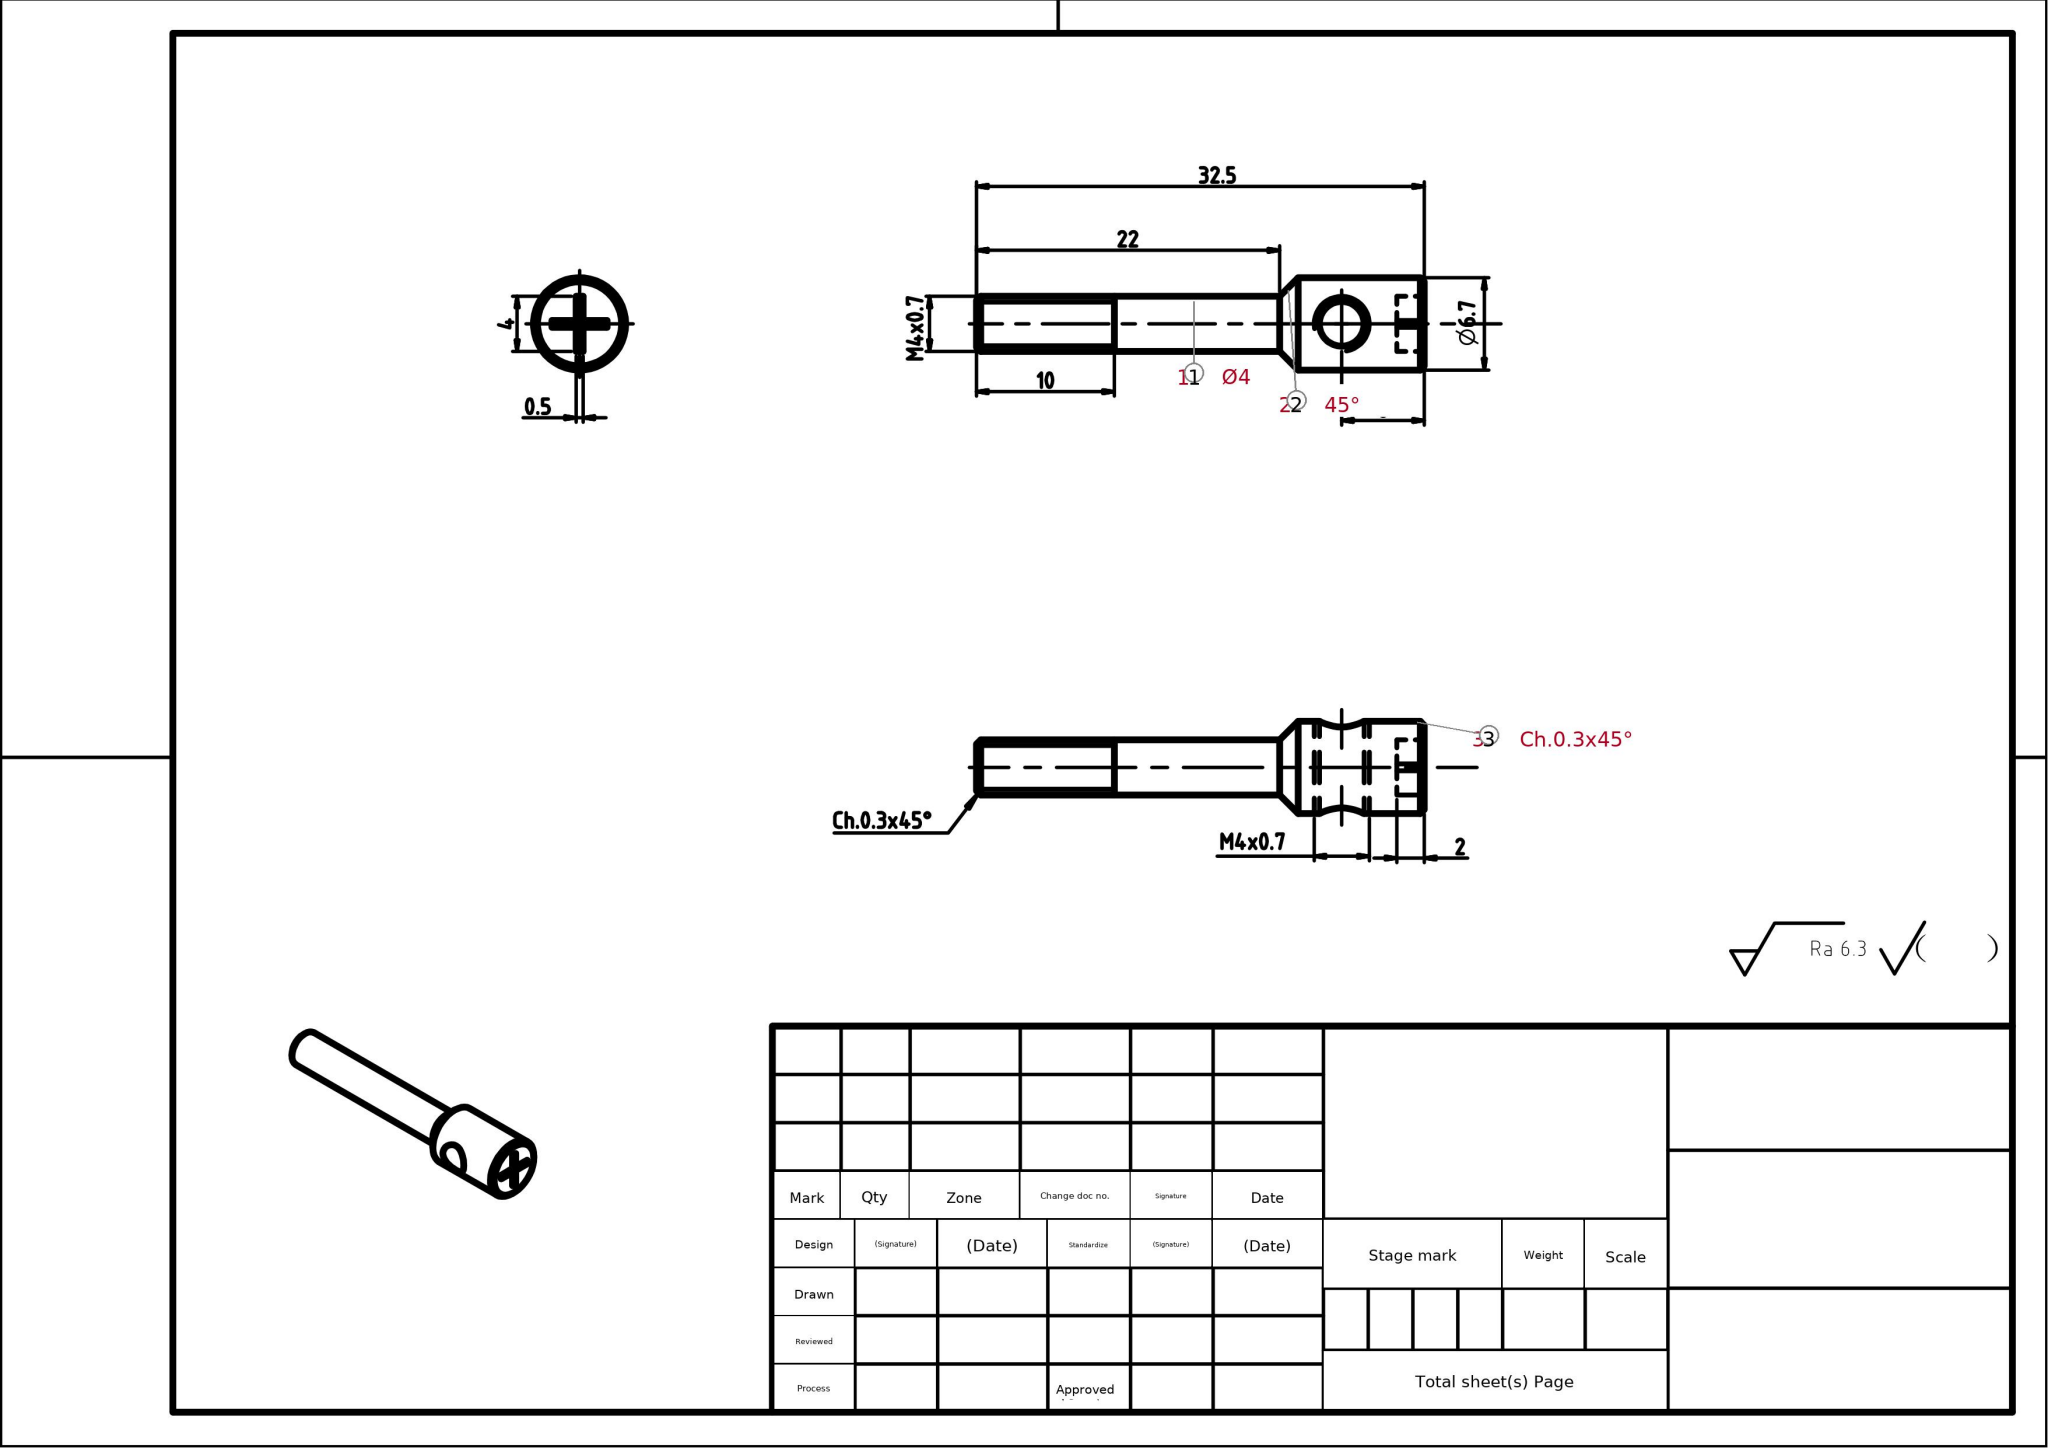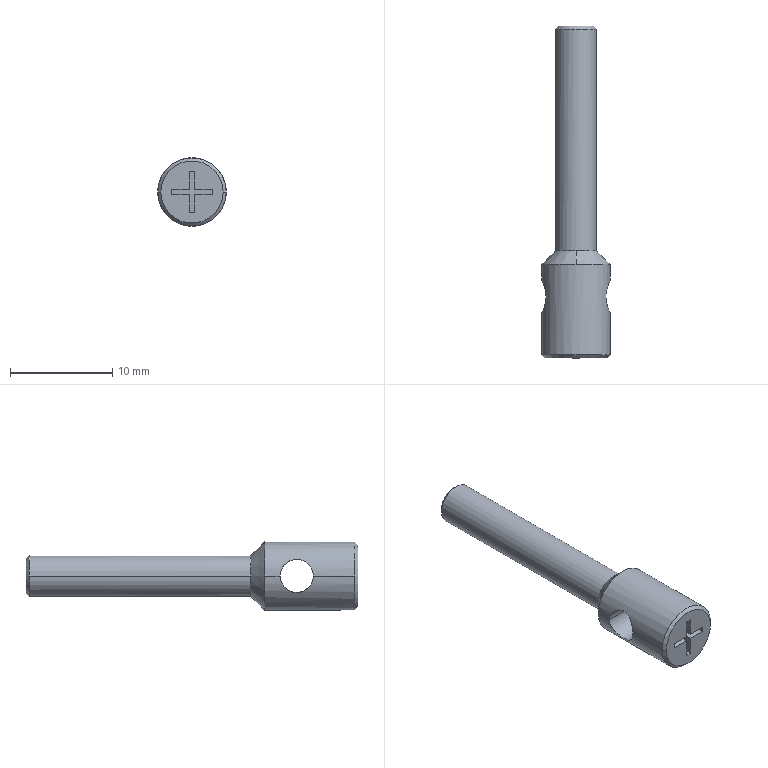Part | SolidWorks | mm | 1 solid | 27 faces | box 6.7 x 32.5 x 6.7 mm | volume 567 mm3 | plane 15 | cone 6 | cylinder 6 | commonest cylinder face diameters 3.242 x2 6.7 x2 4 x2
STEP:
#1=CARTESIAN_POINT('',(0.,10.5,2.));
#2=VERTEX_POINT('',#1);
#3=CARTESIAN_POINT('',(2.,10.5,-0.));
#4=VERTEX_POINT('',#3);
#5=CARTESIAN_POINT('',(0.,10.5,0.));
#6=DIRECTION('',(0.,1.,0.));
#7=DIRECTION('',(-1.,0.,0.));
#8=AXIS2_PLACEMENT_3D('',#5,#6,#7);
#9=CIRCLE('',#8,2.);
#10=EDGE_CURVE('',#2,#4,#9,.T.);
#11=ORIENTED_EDGE('',*,*,#10,.F.);
#12=CARTESIAN_POINT('',(0.,9.15,3.35));
#13=VERTEX_POINT('',#12);
#14=CARTESIAN_POINT('',(0.,9.825,2.675));
#15=DIRECTION('',(0.,-0.7071,0.7071));
#16=VECTOR('',#15,1000.);
#17=LINE('',#14,#16);
#18=EDGE_CURVE('',#2,#13,#17,.T.);
#19=ORIENTED_EDGE('',*,*,#18,.T.);
#20=CARTESIAN_POINT('',(3.35,9.15,0.));
#21=VERTEX_POINT('',#20);
#22=CARTESIAN_POINT('',(0.,9.15,0.));
#23=DIRECTION('',(0.,-1.,0.));
#24=DIRECTION('',(-1.,0.,0.));
#25=AXIS2_PLACEMENT_3D('',#22,#23,#24);
#26=CIRCLE('',#25,3.35);
#27=EDGE_CURVE('',#21,#13,#26,.T.);
#28=ORIENTED_EDGE('',*,*,#27,.F.);
#29=CARTESIAN_POINT('',(0.,9.15,-3.35));
#30=VERTEX_POINT('',#29);
#31=CARTESIAN_POINT('',(0.,9.15,0.));
#32=DIRECTION('',(0.,-1.,0.));
#33=DIRECTION('',(-1.,0.,0.));
#34=AXIS2_PLACEMENT_3D('',#31,#32,#33);
#35=CIRCLE('',#34,3.35);
#36=EDGE_CURVE('',#30,#21,#35,.T.);
#37=ORIENTED_EDGE('',*,*,#36,.F.);
#38=CARTESIAN_POINT('',(0.,10.5,-2.));
#39=VERTEX_POINT('',#38);
#40=CARTESIAN_POINT('',(0.,9.825,-2.675));
#41=DIRECTION('',(0.,-0.7071,-0.7071));
#42=VECTOR('',#41,1000.);
#43=LINE('',#40,#42);
#44=EDGE_CURVE('',#39,#30,#43,.T.);
#45=ORIENTED_EDGE('',*,*,#44,.F.);
#46=CARTESIAN_POINT('',(0.,10.5,0.));
#47=DIRECTION('',(0.,1.,0.));
#48=DIRECTION('',(-1.,0.,0.));
#49=AXIS2_PLACEMENT_3D('',#46,#47,#48);
#50=CIRCLE('',#49,2.);
#51=EDGE_CURVE('',#4,#39,#50,.T.);
#52=ORIENTED_EDGE('',*,*,#51,.F.);
#53=EDGE_LOOP('',(#11,#19,#28,#37,#45,#52));
#54=FACE_OUTER_BOUND('',#53,.T.);
#55=CARTESIAN_POINT('',(0.,9.825,0.));
#56=DIRECTION('',(0.,-1.,0.));
#57=DIRECTION('',(0.,0.,-1.));
#58=AXIS2_PLACEMENT_3D('',#55,#56,#57);
#59=CONICAL_SURFACE('',#58,2.675,0.7854);
#60=ADVANCED_FACE('',(#54),#59,.T.);
#61=CARTESIAN_POINT('',(-3.35,4.379,0.));
#62=VERTEX_POINT('',#61);
#63=CARTESIAN_POINT('',(-3.35,7.621,0.));
#64=VERTEX_POINT('',#63);
#65=CARTESIAN_POINT('',(-3.35,4.379,0.));
#66=CARTESIAN_POINT('',(-3.35,4.379,-0.1079));
#67=CARTESIAN_POINT('',(-3.345,4.389,-0.2144));
#68=CARTESIAN_POINT('',(-3.325,4.431,-0.4232));
#69=CARTESIAN_POINT('',(-3.31,4.463,-0.5273));
#70=CARTESIAN_POINT('',(-3.272,4.546,-0.7243));
#71=CARTESIAN_POINT('',(-3.25,4.596,-0.817));
#72=CARTESIAN_POINT('',(-3.201,4.712,-0.9908));
#73=CARTESIAN_POINT('',(-3.175,4.778,-1.071));
#74=CARTESIAN_POINT('',(-3.12,4.931,-1.224));
#75=CARTESIAN_POINT('',(-3.092,5.013,-1.291));
#76=CARTESIAN_POINT('',(-3.054,5.143,-1.377));
#77=CARTESIAN_POINT('',(-3.042,5.188,-1.404));
#78=CARTESIAN_POINT('',(-3.018,5.28,-1.453));
#79=CARTESIAN_POINT('',(-3.008,5.325,-1.475));
#80=CARTESIAN_POINT('',(-2.955,5.577,-1.58));
#81=CARTESIAN_POINT('',(-2.932,5.786,-1.621));
#82=CARTESIAN_POINT('',(-2.932,6.107,-1.621));
#83=CARTESIAN_POINT('',(-2.937,6.213,-1.611));
#84=CARTESIAN_POINT('',(-2.954,6.369,-1.58));
#85=CARTESIAN_POINT('',(-2.961,6.42,-1.567));
#86=CARTESIAN_POINT('',(-2.978,6.523,-1.535));
#87=CARTESIAN_POINT('',(-2.987,6.576,-1.516));
#88=CARTESIAN_POINT('',(-3.018,6.721,-1.455));
#89=CARTESIAN_POINT('',(-3.041,6.813,-1.406));
#90=CARTESIAN_POINT('',(-3.092,6.987,-1.291));
#91=CARTESIAN_POINT('',(-3.12,7.07,-1.223));
#92=CARTESIAN_POINT('',(-3.175,7.221,-1.072));
#93=CARTESIAN_POINT('',(-3.201,7.288,-0.9909));
#94=CARTESIAN_POINT('',(-3.25,7.404,-0.8171));
#95=CARTESIAN_POINT('',(-3.272,7.453,-0.7259));
#96=CARTESIAN_POINT('',(-3.329,7.579,-0.4256));
#97=CARTESIAN_POINT('',(-3.35,7.621,-0.2159));
#98=CARTESIAN_POINT('',(-3.35,7.621,0.));
#99=B_SPLINE_CURVE_WITH_KNOTS('',3,(#65,#66,#67,#68,#69,#70,#71,#72,#73,#74,#75,#76,#77,#78,#79,#80,#81,#82,#83,#84,#85,#86,#87,#88,#89,#90,#91,#92,#93,#94,#95,#96,#97,#98),.UNSPECIFIED.,.F.,.F.,(4,2,2,2,2,2,2,2,2,2,2,2,2,2,2,2,4),(0.,0.0625,0.125,0.1875,0.25,0.3125,0.3438,0.375,0.5,0.5625,0.5938,0.625,0.6875,0.75,0.8125,0.875,1.),.UNSPECIFIED.);
#100=EDGE_CURVE('',#62,#64,#99,.T.);
#101=ORIENTED_EDGE('',*,*,#100,.F.);
#102=CARTESIAN_POINT('',(3.35,4.379,-0.));
#103=VERTEX_POINT('',#102);
#104=CARTESIAN_POINT('',(30.503,4.379,0.));
#105=DIRECTION('',(1.,0.,0.));
#106=VECTOR('',#105,1000.);
#107=LINE('',#104,#106);
#108=EDGE_CURVE('',#62,#103,#107,.T.);
#109=ORIENTED_EDGE('',*,*,#108,.T.);
#110=CARTESIAN_POINT('',(2.932,6.,-1.621));
#111=VERTEX_POINT('',#110);
#112=CARTESIAN_POINT('',(2.932,6.,-1.621));
#113=CARTESIAN_POINT('',(2.932,5.893,-1.621));
#114=CARTESIAN_POINT('',(2.937,5.787,-1.611));
#115=CARTESIAN_POINT('',(2.954,5.631,-1.58));
#116=CARTESIAN_POINT('',(2.961,5.579,-1.567));
#117=CARTESIAN_POINT('',(2.978,5.477,-1.535));
#118=CARTESIAN_POINT('',(2.987,5.424,-1.516));
#119=CARTESIAN_POINT('',(3.018,5.279,-1.455));
#120=CARTESIAN_POINT('',(3.041,5.187,-1.406));
#121=CARTESIAN_POINT('',(3.092,5.013,-1.291));
#122=CARTESIAN_POINT('',(3.12,4.93,-1.223));
#123=CARTESIAN_POINT('',(3.175,4.779,-1.072));
#124=CARTESIAN_POINT('',(3.201,4.712,-0.9909));
#125=CARTESIAN_POINT('',(3.25,4.596,-0.8171));
#126=CARTESIAN_POINT('',(3.272,4.547,-0.7259));
#127=CARTESIAN_POINT('',(3.329,4.421,-0.4256));
#128=CARTESIAN_POINT('',(3.35,4.379,-0.2159));
#129=CARTESIAN_POINT('',(3.35,4.379,-0.));
#130=B_SPLINE_CURVE_WITH_KNOTS('',3,(#112,#113,#114,#115,#116,#117,#118,#119,#120,#121,#122,#123,#124,#125,#126,#127,#128,#129),.UNSPECIFIED.,.F.,.F.,(4,2,2,2,2,2,2,2,4),(0.,0.125,0.1875,0.25,0.375,0.5,0.625,0.75,1.),.UNSPECIFIED.);
#131=EDGE_CURVE('',#111,#103,#130,.T.);
#132=ORIENTED_EDGE('',*,*,#131,.F.);
#133=CARTESIAN_POINT('',(3.35,7.621,-0.));
#134=VERTEX_POINT('',#133);
#135=CARTESIAN_POINT('',(3.35,7.621,-0.));
#136=CARTESIAN_POINT('',(3.35,7.621,-0.1079));
#137=CARTESIAN_POINT('',(3.345,7.611,-0.2144));
#138=CARTESIAN_POINT('',(3.325,7.569,-0.4232));
#139=CARTESIAN_POINT('',(3.31,7.537,-0.5273));
#140=CARTESIAN_POINT('',(3.272,7.454,-0.7243));
#141=CARTESIAN_POINT('',(3.25,7.404,-0.817));
#142=CARTESIAN_POINT('',(3.201,7.288,-0.9908));
#143=CARTESIAN_POINT('',(3.175,7.222,-1.071));
#144=CARTESIAN_POINT('',(3.12,7.069,-1.224));
#145=CARTESIAN_POINT('',(3.092,6.987,-1.291));
#146=CARTESIAN_POINT('',(3.054,6.857,-1.377));
#147=CARTESIAN_POINT('',(3.042,6.812,-1.404));
#148=CARTESIAN_POINT('',(3.018,6.72,-1.453));
#149=CARTESIAN_POINT('',(3.008,6.675,-1.475));
#150=CARTESIAN_POINT('',(2.955,6.423,-1.58));
#151=CARTESIAN_POINT('',(2.932,6.215,-1.621));
#152=CARTESIAN_POINT('',(2.932,6.,-1.621));
#153=B_SPLINE_CURVE_WITH_KNOTS('',3,(#135,#136,#137,#138,#139,#140,#141,#142,#143,#144,#145,#146,#147,#148,#149,#150,#151,#152),.UNSPECIFIED.,.F.,.F.,(4,2,2,2,2,2,2,2,4),(0.,0.125,0.25,0.375,0.5,0.625,0.6875,0.75,1.),.UNSPECIFIED.);
#154=EDGE_CURVE('',#134,#111,#153,.T.);
#155=ORIENTED_EDGE('',*,*,#154,.F.);
#156=CARTESIAN_POINT('',(30.503,7.621,0.));
#157=DIRECTION('',(1.,0.,0.));
#158=VECTOR('',#157,1000.);
#159=LINE('',#156,#158);
#160=EDGE_CURVE('',#64,#134,#159,.T.);
#161=ORIENTED_EDGE('',*,*,#160,.F.);
#162=EDGE_LOOP('',(#101,#109,#132,#155,#161));
#163=FACE_OUTER_BOUND('',#162,.T.);
#164=CARTESIAN_POINT('',(30.503,6.,0.));
#165=DIRECTION('',(1.,0.,0.));
#166=DIRECTION('',(0.,1.,0.));
#167=AXIS2_PLACEMENT_3D('',#164,#165,#166);
#168=CYLINDRICAL_SURFACE('',#167,1.621);
#169=ADVANCED_FACE('',(#163),#168,.F.);
#170=CARTESIAN_POINT('',(3.35,0.3,0.));
#171=VERTEX_POINT('',#170);
#172=CARTESIAN_POINT('',(-3.35,0.3,-0.));
#173=VERTEX_POINT('',#172);
#174=CARTESIAN_POINT('',(0.,0.3,0.));
#175=DIRECTION('',(0.,-1.,0.));
#176=DIRECTION('',(1.,0.,0.));
#177=AXIS2_PLACEMENT_3D('',#174,#175,#176);
#178=CIRCLE('',#177,3.35);
#179=EDGE_CURVE('',#171,#173,#178,.T.);
#180=ORIENTED_EDGE('',*,*,#179,.F.);
#181=CARTESIAN_POINT('',(3.35,0.,0.));
#182=DIRECTION('',(0.,1.,0.));
#183=VECTOR('',#182,1000.);
#184=LINE('',#181,#183);
#185=EDGE_CURVE('',#171,#103,#184,.T.);
#186=ORIENTED_EDGE('',*,*,#185,.T.);
#187=CARTESIAN_POINT('',(3.35,4.379,-0.));
#188=CARTESIAN_POINT('',(3.35,4.379,0.1079));
#189=CARTESIAN_POINT('',(3.345,4.389,0.2144));
#190=CARTESIAN_POINT('',(3.325,4.431,0.4232));
#191=CARTESIAN_POINT('',(3.31,4.463,0.5273));
#192=CARTESIAN_POINT('',(3.272,4.546,0.7243));
#193=CARTESIAN_POINT('',(3.25,4.596,0.817));
#194=CARTESIAN_POINT('',(3.201,4.712,0.9908));
#195=CARTESIAN_POINT('',(3.175,4.778,1.071));
#196=CARTESIAN_POINT('',(3.12,4.931,1.224));
#197=CARTESIAN_POINT('',(3.092,5.013,1.291));
#198=CARTESIAN_POINT('',(3.054,5.143,1.377));
#199=CARTESIAN_POINT('',(3.042,5.188,1.404));
#200=CARTESIAN_POINT('',(3.018,5.28,1.453));
#201=CARTESIAN_POINT('',(3.008,5.325,1.475));
#202=CARTESIAN_POINT('',(2.955,5.577,1.58));
#203=CARTESIAN_POINT('',(2.932,5.786,1.621));
#204=CARTESIAN_POINT('',(2.932,6.107,1.621));
#205=CARTESIAN_POINT('',(2.937,6.213,1.611));
#206=CARTESIAN_POINT('',(2.954,6.369,1.58));
#207=CARTESIAN_POINT('',(2.961,6.42,1.567));
#208=CARTESIAN_POINT('',(2.978,6.523,1.535));
#209=CARTESIAN_POINT('',(2.987,6.576,1.516));
#210=CARTESIAN_POINT('',(3.018,6.721,1.455));
#211=CARTESIAN_POINT('',(3.041,6.813,1.406));
#212=CARTESIAN_POINT('',(3.092,6.987,1.291));
#213=CARTESIAN_POINT('',(3.12,7.07,1.223));
#214=CARTESIAN_POINT('',(3.175,7.221,1.072));
#215=CARTESIAN_POINT('',(3.201,7.288,0.9909));
#216=CARTESIAN_POINT('',(3.25,7.404,0.8171));
#217=CARTESIAN_POINT('',(3.272,7.453,0.7259));
#218=CARTESIAN_POINT('',(3.329,7.579,0.4256));
#219=CARTESIAN_POINT('',(3.35,7.621,0.2159));
#220=CARTESIAN_POINT('',(3.35,7.621,-0.));
#221=B_SPLINE_CURVE_WITH_KNOTS('',3,(#187,#188,#189,#190,#191,#192,#193,#194,#195,#196,#197,#198,#199,#200,#201,#202,#203,#204,#205,#206,#207,#208,#209,#210,#211,#212,#213,#214,#215,#216,#217,#218,#219,#220),.UNSPECIFIED.,.F.,.F.,(4,2,2,2,2,2,2,2,2,2,2,2,2,2,2,2,4),(0.,0.0625,0.125,0.1875,0.25,0.3125,0.3437,0.375,0.5,0.5625,0.5937,0.625,0.6875,0.75,0.8125,0.875,1.),.UNSPECIFIED.);
#222=EDGE_CURVE('',#103,#134,#221,.T.);
#223=ORIENTED_EDGE('',*,*,#222,.T.);
#224=CARTESIAN_POINT('',(3.35,0.,0.));
#225=DIRECTION('',(0.,1.,0.));
#226=VECTOR('',#225,1000.);
#227=LINE('',#224,#226);
#228=EDGE_CURVE('',#134,#21,#227,.T.);
#229=ORIENTED_EDGE('',*,*,#228,.T.);
#230=ORIENTED_EDGE('',*,*,#27,.T.);
#231=CARTESIAN_POINT('',(-3.35,9.15,0.));
#232=VERTEX_POINT('',#231);
#233=CARTESIAN_POINT('',(0.,9.15,0.));
#234=DIRECTION('',(0.,-1.,0.));
#235=DIRECTION('',(-1.,0.,0.));
#236=AXIS2_PLACEMENT_3D('',#233,#234,#235);
#237=CIRCLE('',#236,3.35);
#238=EDGE_CURVE('',#13,#232,#237,.T.);
#239=ORIENTED_EDGE('',*,*,#238,.T.);
#240=CARTESIAN_POINT('',(-3.35,0.,0.));
#241=DIRECTION('',(0.,1.,0.));
#242=VECTOR('',#241,1000.);
#243=LINE('',#240,#242);
#244=EDGE_CURVE('',#64,#232,#243,.T.);
#245=ORIENTED_EDGE('',*,*,#244,.F.);
#246=CARTESIAN_POINT('',(-3.35,7.621,0.));
#247=CARTESIAN_POINT('',(-3.35,7.621,0.1079));
#248=CARTESIAN_POINT('',(-3.345,7.611,0.2144));
#249=CARTESIAN_POINT('',(-3.325,7.569,0.4232));
#250=CARTESIAN_POINT('',(-3.31,7.537,0.5273));
#251=CARTESIAN_POINT('',(-3.272,7.454,0.7243));
#252=CARTESIAN_POINT('',(-3.25,7.404,0.817));
#253=CARTESIAN_POINT('',(-3.201,7.288,0.9908));
#254=CARTESIAN_POINT('',(-3.175,7.222,1.071));
#255=CARTESIAN_POINT('',(-3.12,7.069,1.224));
#256=CARTESIAN_POINT('',(-3.092,6.987,1.291));
#257=CARTESIAN_POINT('',(-3.054,6.857,1.377));
#258=CARTESIAN_POINT('',(-3.042,6.812,1.404));
#259=CARTESIAN_POINT('',(-3.018,6.72,1.453));
#260=CARTESIAN_POINT('',(-3.008,6.675,1.475));
#261=CARTESIAN_POINT('',(-2.955,6.423,1.58));
#262=CARTESIAN_POINT('',(-2.932,6.214,1.621));
#263=CARTESIAN_POINT('',(-2.932,5.893,1.621));
#264=CARTESIAN_POINT('',(-2.937,5.787,1.611));
#265=CARTESIAN_POINT('',(-2.954,5.631,1.58));
#266=CARTESIAN_POINT('',(-2.961,5.58,1.567));
#267=CARTESIAN_POINT('',(-2.978,5.477,1.535));
#268=CARTESIAN_POINT('',(-2.987,5.424,1.516));
#269=CARTESIAN_POINT('',(-3.018,5.279,1.455));
#270=CARTESIAN_POINT('',(-3.041,5.187,1.406));
#271=CARTESIAN_POINT('',(-3.092,5.013,1.291));
#272=CARTESIAN_POINT('',(-3.12,4.93,1.223));
#273=CARTESIAN_POINT('',(-3.175,4.779,1.072));
#274=CARTESIAN_POINT('',(-3.201,4.712,0.9909));
#275=CARTESIAN_POINT('',(-3.25,4.596,0.8171));
#276=CARTESIAN_POINT('',(-3.272,4.547,0.7259));
#277=CARTESIAN_POINT('',(-3.329,4.421,0.4256));
#278=CARTESIAN_POINT('',(-3.35,4.379,0.2159));
#279=CARTESIAN_POINT('',(-3.35,4.379,0.));
#280=B_SPLINE_CURVE_WITH_KNOTS('',3,(#246,#247,#248,#249,#250,#251,#252,#253,#254,#255,#256,#257,#258,#259,#260,#261,#262,#263,#264,#265,#266,#267,#268,#269,#270,#271,#272,#273,#274,#275,#276,#277,#278,#279),.UNSPECIFIED.,.F.,.F.,(4,2,2,2,2,2,2,2,2,2,2,2,2,2,2,2,4),(0.,0.0625,0.125,0.1875,0.25,0.3125,0.3438,0.375,0.5,0.5625,0.5938,0.625,0.6875,0.75,0.8125,0.875,1.),.UNSPECIFIED.);
#281=EDGE_CURVE('',#64,#62,#280,.T.);
#282=ORIENTED_EDGE('',*,*,#281,.T.);
#283=CARTESIAN_POINT('',(-3.35,0.,0.));
#284=DIRECTION('',(0.,1.,0.));
#285=VECTOR('',#284,1000.);
#286=LINE('',#283,#285);
#287=EDGE_CURVE('',#173,#62,#286,.T.);
#288=ORIENTED_EDGE('',*,*,#287,.F.);
#289=EDGE_LOOP('',(#180,#186,#223,#229,#230,#239,#245,#282,#288));
#290=FACE_OUTER_BOUND('',#289,.T.);
#291=CARTESIAN_POINT('',(0.,0.,0.));
#292=DIRECTION('',(0.,1.,0.));
#293=DIRECTION('',(-1.,0.,0.));
#294=AXIS2_PLACEMENT_3D('',#291,#292,#293);
#295=CYLINDRICAL_SURFACE('',#294,3.35);
#296=ADVANCED_FACE('',(#290),#295,.T.);
#297=CARTESIAN_POINT('',(3.05,0.,0.));
#298=VERTEX_POINT('',#297);
#299=CARTESIAN_POINT('',(-3.05,0.,-0.));
#300=VERTEX_POINT('',#299);
#301=CARTESIAN_POINT('',(0.,0.,0.));
#302=DIRECTION('',(0.,1.,0.));
#303=DIRECTION('',(1.,0.,0.));
#304=AXIS2_PLACEMENT_3D('',#301,#302,#303);
#305=CIRCLE('',#304,3.05);
#306=EDGE_CURVE('',#298,#300,#305,.T.);
#307=ORIENTED_EDGE('',*,*,#306,.T.);
#308=CARTESIAN_POINT('',(-3.2,0.15,-0.));
#309=DIRECTION('',(-0.7071,0.7071,-0.));
#310=VECTOR('',#309,1000.);
#311=LINE('',#308,#310);
#312=EDGE_CURVE('',#300,#173,#311,.T.);
#313=ORIENTED_EDGE('',*,*,#312,.T.);
#314=CARTESIAN_POINT('',(0.,0.3,0.));
#315=DIRECTION('',(0.,-1.,0.));
#316=DIRECTION('',(1.,0.,0.));
#317=AXIS2_PLACEMENT_3D('',#314,#315,#316);
#318=CIRCLE('',#317,3.35);
#319=EDGE_CURVE('',#173,#171,#318,.T.);
#320=ORIENTED_EDGE('',*,*,#319,.T.);
#321=CARTESIAN_POINT('',(3.2,0.15,0.));
#322=DIRECTION('',(0.7071,0.7071,0.));
#323=VECTOR('',#322,1000.);
#324=LINE('',#321,#323);
#325=EDGE_CURVE('',#298,#171,#324,.T.);
#326=ORIENTED_EDGE('',*,*,#325,.F.);
#327=EDGE_LOOP('',(#307,#313,#320,#326));
#328=FACE_OUTER_BOUND('',#327,.T.);
#329=CARTESIAN_POINT('',(0.,0.15,0.));
#330=DIRECTION('',(0.,1.,0.));
#331=DIRECTION('',(1.,0.,0.));
#332=AXIS2_PLACEMENT_3D('',#329,#330,#331);
#333=CONICAL_SURFACE('',#332,3.2,0.7854);
#334=ADVANCED_FACE('',(#328),#333,.T.);
#335=CARTESIAN_POINT('',(2.,32.2,-0.));
#336=VERTEX_POINT('',#335);
#337=CARTESIAN_POINT('',(-2.,32.2,0.));
#338=VERTEX_POINT('',#337);
#339=CARTESIAN_POINT('',(0.,32.2,0.));
#340=DIRECTION('',(0.,1.,0.));
#341=DIRECTION('',(-1.,0.,0.));
#342=AXIS2_PLACEMENT_3D('',#339,#340,#341);
#343=CIRCLE('',#342,2.);
#344=EDGE_CURVE('',#336,#338,#343,.T.);
#345=ORIENTED_EDGE('',*,*,#344,.F.);
#346=CARTESIAN_POINT('',(2.,32.5,-0.));
#347=DIRECTION('',(0.,-1.,0.));
#348=VECTOR('',#347,1000.);
#349=LINE('',#346,#348);
#350=EDGE_CURVE('',#336,#4,#349,.T.);
#351=ORIENTED_EDGE('',*,*,#350,.T.);
#352=ORIENTED_EDGE('',*,*,#51,.T.);
#353=CARTESIAN_POINT('',(-2.,10.5,0.));
#354=VERTEX_POINT('',#353);
#355=CARTESIAN_POINT('',(0.,10.5,0.));
#356=DIRECTION('',(0.,1.,0.));
#357=DIRECTION('',(-1.,0.,0.));
#358=AXIS2_PLACEMENT_3D('',#355,#356,#357);
#359=CIRCLE('',#358,2.);
#360=EDGE_CURVE('',#39,#354,#359,.T.);
#361=ORIENTED_EDGE('',*,*,#360,.T.);
#362=CARTESIAN_POINT('',(-2.,32.5,0.));
#363=DIRECTION('',(0.,-1.,0.));
#364=VECTOR('',#363,1000.);
#365=LINE('',#362,#364);
#366=EDGE_CURVE('',#338,#354,#365,.T.);
#367=ORIENTED_EDGE('',*,*,#366,.F.);
#368=EDGE_LOOP('',(#345,#351,#352,#361,#367));
#369=FACE_OUTER_BOUND('',#368,.T.);
#370=CARTESIAN_POINT('',(0.,32.5,0.));
#371=DIRECTION('',(0.,-1.,0.));
#372=DIRECTION('',(-1.,0.,0.));
#373=AXIS2_PLACEMENT_3D('',#370,#371,#372);
#374=CYLINDRICAL_SURFACE('',#373,2.);
#375=ADVANCED_FACE('',(#369),#374,.T.);
#376=CARTESIAN_POINT('',(-1.7,32.5,0.));
#377=VERTEX_POINT('',#376);
#378=CARTESIAN_POINT('',(1.7,32.5,-0.));
#379=VERTEX_POINT('',#378);
#380=CARTESIAN_POINT('',(0.,32.5,0.));
#381=DIRECTION('',(0.,-1.,0.));
#382=DIRECTION('',(-1.,0.,0.));
#383=AXIS2_PLACEMENT_3D('',#380,#381,#382);
#384=CIRCLE('',#383,1.7);
#385=EDGE_CURVE('',#377,#379,#384,.T.);
#386=ORIENTED_EDGE('',*,*,#385,.T.);
#387=CARTESIAN_POINT('',(1.85,32.35,-0.));
#388=DIRECTION('',(0.7071,-0.7071,-0.));
#389=VECTOR('',#388,1000.);
#390=LINE('',#387,#389);
#391=EDGE_CURVE('',#379,#336,#390,.T.);
#392=ORIENTED_EDGE('',*,*,#391,.T.);
#393=ORIENTED_EDGE('',*,*,#344,.T.);
#394=CARTESIAN_POINT('',(-1.85,32.35,0.));
#395=DIRECTION('',(-0.7071,-0.7071,0.));
#396=VECTOR('',#395,1000.);
#397=LINE('',#394,#396);
#398=EDGE_CURVE('',#377,#338,#397,.T.);
#399=ORIENTED_EDGE('',*,*,#398,.F.);
#400=EDGE_LOOP('',(#386,#392,#393,#399));
#401=FACE_OUTER_BOUND('',#400,.T.);
#402=CARTESIAN_POINT('',(0.,32.35,0.));
#403=DIRECTION('',(0.,-1.,0.));
#404=DIRECTION('',(-1.,0.,0.));
#405=AXIS2_PLACEMENT_3D('',#402,#403,#404);
#406=CONICAL_SURFACE('',#405,1.85,0.7854);
#407=ADVANCED_FACE('',(#401),#406,.T.);
#408=CARTESIAN_POINT('',(0.25,0.,0.25));
#409=VERTEX_POINT('',#408);
#410=CARTESIAN_POINT('',(0.25,2.,0.25));
#411=VERTEX_POINT('',#410);
#412=CARTESIAN_POINT('',(0.25,0.,0.25));
#413=DIRECTION('',(0.,1.,0.));
#414=VECTOR('',#413,1000.);
#415=LINE('',#412,#414);
#416=EDGE_CURVE('',#409,#411,#415,.T.);
#417=ORIENTED_EDGE('',*,*,#416,.F.);
#418=CARTESIAN_POINT('',(0.25,0.,2.));
#419=VERTEX_POINT('',#418);
#420=CARTESIAN_POINT('',(0.25,0.,1.));
#421=DIRECTION('',(0.,0.,-1.));
#422=VECTOR('',#421,1000.);
#423=LINE('',#420,#422);
#424=EDGE_CURVE('',#419,#409,#423,.T.);
#425=ORIENTED_EDGE('',*,*,#424,.F.);
#426=CARTESIAN_POINT('',(0.25,2.,2.));
#427=VERTEX_POINT('',#426);
#428=CARTESIAN_POINT('',(0.25,0.,2.));
#429=DIRECTION('',(0.,1.,0.));
#430=VECTOR('',#429,1000.);
#431=LINE('',#428,#430);
#432=EDGE_CURVE('',#419,#427,#431,.T.);
#433=ORIENTED_EDGE('',*,*,#432,.T.);
#434=CARTESIAN_POINT('',(0.25,2.,-2.));
#435=DIRECTION('',(0.,0.,-1.));
#436=VECTOR('',#435,1000.);
#437=LINE('',#434,#436);
#438=EDGE_CURVE('',#427,#411,#437,.T.);
#439=ORIENTED_EDGE('',*,*,#438,.T.);
#440=EDGE_LOOP('',(#417,#425,#433,#439));
#441=FACE_OUTER_BOUND('',#440,.T.);
#442=CARTESIAN_POINT('',(0.25,0.,2.));
#443=DIRECTION('',(1.,0.,0.));
#444=DIRECTION('',(0.,-0.,1.));
#445=AXIS2_PLACEMENT_3D('',#442,#443,#444);
#446=PLANE('',#445);
#447=ADVANCED_FACE('',(#441),#446,.F.);
#448=CARTESIAN_POINT('',(-0.25,2.,0.25));
#449=VERTEX_POINT('',#448);
#450=CARTESIAN_POINT('',(-0.25,0.,0.25));
#451=VERTEX_POINT('',#450);
#452=CARTESIAN_POINT('',(-0.25,0.,0.25));
#453=DIRECTION('',(0.,-1.,0.));
#454=VECTOR('',#453,1000.);
#455=LINE('',#452,#454);
#456=EDGE_CURVE('',#449,#451,#455,.T.);
#457=ORIENTED_EDGE('',*,*,#456,.F.);
#458=CARTESIAN_POINT('',(-0.25,2.,2.));
#459=VERTEX_POINT('',#458);
#460=CARTESIAN_POINT('',(-0.25,2.,2.));
#461=DIRECTION('',(-0.,0.,1.));
#462=VECTOR('',#461,1000.);
#463=LINE('',#460,#462);
#464=EDGE_CURVE('',#449,#459,#463,.T.);
#465=ORIENTED_EDGE('',*,*,#464,.T.);
#466=CARTESIAN_POINT('',(-0.25,0.,2.));
#467=VERTEX_POINT('',#466);
#468=CARTESIAN_POINT('',(-0.25,0.,2.));
#469=DIRECTION('',(0.,1.,0.));
#470=VECTOR('',#469,1000.);
#471=LINE('',#468,#470);
#472=EDGE_CURVE('',#467,#459,#471,.T.);
#473=ORIENTED_EDGE('',*,*,#472,.F.);
#474=CARTESIAN_POINT('',(-0.25,0.,-1.));
#475=DIRECTION('',(-0.,0.,1.));
#476=VECTOR('',#475,1000.);
#477=LINE('',#474,#476);
#478=EDGE_CURVE('',#451,#467,#477,.T.);
#479=ORIENTED_EDGE('',*,*,#478,.F.);
#480=EDGE_LOOP('',(#457,#465,#473,#479));
#481=FACE_OUTER_BOUND('',#480,.T.);
#482=CARTESIAN_POINT('',(-0.25,0.,-2.));
#483=DIRECTION('',(-1.,0.,-0.));
#484=DIRECTION('',(-0.,0.,1.));
#485=AXIS2_PLACEMENT_3D('',#482,#483,#484);
#486=PLANE('',#485);
#487=ADVANCED_FACE('',(#481),#486,.F.);
#488=CARTESIAN_POINT('',(0.25,0.,-2.));
#489=VERTEX_POINT('',#488);
#490=CARTESIAN_POINT('',(-0.25,0.,-2.));
#491=VERTEX_POINT('',#490);
#492=CARTESIAN_POINT('',(0.125,0.,-2.));
#493=DIRECTION('',(-1.,0.,-0.));
#494=VECTOR('',#493,1000.);
#495=LINE('',#492,#494);
#496=EDGE_CURVE('',#489,#491,#495,.T.);
#497=ORIENTED_EDGE('',*,*,#496,.F.);
#498=CARTESIAN_POINT('',(0.25,2.,-2.));
#499=VERTEX_POINT('',#498);
#500=CARTESIAN_POINT('',(0.25,0.,-2.));
#501=DIRECTION('',(0.,1.,0.));
#502=VECTOR('',#501,1000.);
#503=LINE('',#500,#502);
#504=EDGE_CURVE('',#489,#499,#503,.T.);
#505=ORIENTED_EDGE('',*,*,#504,.T.);
#506=CARTESIAN_POINT('',(-0.25,2.,-2.));
#507=VERTEX_POINT('',#506);
#508=CARTESIAN_POINT('',(-0.25,2.,-2.));
#509=DIRECTION('',(-1.,0.,-0.));
#510=VECTOR('',#509,1000.);
#511=LINE('',#508,#510);
#512=EDGE_CURVE('',#499,#507,#511,.T.);
#513=ORIENTED_EDGE('',*,*,#512,.T.);
#514=CARTESIAN_POINT('',(-0.25,0.,-2.));
#515=DIRECTION('',(0.,1.,0.));
#516=VECTOR('',#515,1000.);
#517=LINE('',#514,#516);
#518=EDGE_CURVE('',#491,#507,#517,.T.);
#519=ORIENTED_EDGE('',*,*,#518,.F.);
#520=EDGE_LOOP('',(#497,#505,#513,#519));
#521=FACE_OUTER_BOUND('',#520,.T.);
#522=CARTESIAN_POINT('',(0.25,0.,-2.));
#523=DIRECTION('',(0.,0.,-1.));
#524=DIRECTION('',(0.,-1.,0.));
#525=AXIS2_PLACEMENT_3D('',#522,#523,#524);
#526=PLANE('',#525);
#527=ADVANCED_FACE('',(#521),#526,.F.);
#528=CARTESIAN_POINT('',(0.25,2.,-0.25));
#529=VERTEX_POINT('',#528);
#530=CARTESIAN_POINT('',(0.25,0.,-0.25));
#531=VERTEX_POINT('',#530);
#532=CARTESIAN_POINT('',(0.25,0.,-0.25));
#533=DIRECTION('',(0.,-1.,0.));
#534=VECTOR('',#533,1000.);
#535=LINE('',#532,#534);
#536=EDGE_CURVE('',#529,#531,#535,.T.);
#537=ORIENTED_EDGE('',*,*,#536,.F.);
#538=CARTESIAN_POINT('',(0.25,2.,-2.));
#539=DIRECTION('',(0.,0.,-1.));
#540=VECTOR('',#539,1000.);
#541=LINE('',#538,#540);
#542=EDGE_CURVE('',#529,#499,#541,.T.);
#543=ORIENTED_EDGE('',*,*,#542,.T.);
#544=ORIENTED_EDGE('',*,*,#504,.F.);
#545=CARTESIAN_POINT('',(0.25,0.,1.));
#546=DIRECTION('',(0.,0.,-1.));
#547=VECTOR('',#546,1000.);
#548=LINE('',#545,#547);
#549=EDGE_CURVE('',#531,#489,#548,.T.);
#550=ORIENTED_EDGE('',*,*,#549,.F.);
#551=EDGE_LOOP('',(#537,#543,#544,#550));
#552=FACE_OUTER_BOUND('',#551,.T.);
#553=CARTESIAN_POINT('',(0.25,0.,2.));
#554=DIRECTION('',(1.,0.,0.));
#555=DIRECTION('',(0.,-0.,1.));
#556=AXIS2_PLACEMENT_3D('',#553,#554,#555);
#557=PLANE('',#556);
#558=ADVANCED_FACE('',(#552),#557,.F.);
#559=CARTESIAN_POINT('',(-0.125,0.,2.));
#560=DIRECTION('',(1.,0.,0.));
#561=VECTOR('',#560,1000.);
#562=LINE('',#559,#561);
#563=EDGE_CURVE('',#467,#419,#562,.T.);
#564=ORIENTED_EDGE('',*,*,#563,.F.);
#565=ORIENTED_EDGE('',*,*,#472,.T.);
#566=CARTESIAN_POINT('',(0.25,2.,2.));
#567=DIRECTION('',(1.,0.,0.));
#568=VECTOR('',#567,1000.);
#569=LINE('',#566,#568);
#570=EDGE_CURVE('',#459,#427,#569,.T.);
#571=ORIENTED_EDGE('',*,*,#570,.T.);
#572=ORIENTED_EDGE('',*,*,#432,.F.);
#573=EDGE_LOOP('',(#564,#565,#571,#572));
#574=FACE_OUTER_BOUND('',#573,.T.);
#575=CARTESIAN_POINT('',(-0.25,0.,2.));
#576=DIRECTION('',(-0.,0.,1.));
#577=DIRECTION('',(1.,0.,0.));
#578=AXIS2_PLACEMENT_3D('',#575,#576,#577);
#579=PLANE('',#578);
#580=ADVANCED_FACE('',(#574),#579,.F.);
#581=CARTESIAN_POINT('',(-0.25,0.,-0.25));
#582=VERTEX_POINT('',#581);
#583=CARTESIAN_POINT('',(-0.25,2.,-0.25));
#584=VERTEX_POINT('',#583);
#585=CARTESIAN_POINT('',(-0.25,0.,-0.25));
#586=DIRECTION('',(0.,1.,0.));
#587=VECTOR('',#586,1000.);
#588=LINE('',#585,#587);
#589=EDGE_CURVE('',#582,#584,#588,.T.);
#590=ORIENTED_EDGE('',*,*,#589,.F.);
#591=CARTESIAN_POINT('',(-0.25,0.,-1.));
#592=DIRECTION('',(-0.,0.,1.));
#593=VECTOR('',#592,1000.);
#594=LINE('',#591,#593);
#595=EDGE_CURVE('',#491,#582,#594,.T.);
#596=ORIENTED_EDGE('',*,*,#595,.F.);
#597=ORIENTED_EDGE('',*,*,#518,.T.);
#598=CARTESIAN_POINT('',(-0.25,2.,2.));
#599=DIRECTION('',(-0.,0.,1.));
#600=VECTOR('',#599,1000.);
#601=LINE('',#598,#600);
#602=EDGE_CURVE('',#507,#584,#601,.T.);
#603=ORIENTED_EDGE('',*,*,#602,.T.);
#604=EDGE_LOOP('',(#590,#596,#597,#603));
#605=FACE_OUTER_BOUND('',#604,.T.);
#606=CARTESIAN_POINT('',(-0.25,0.,-2.));
#607=DIRECTION('',(-1.,0.,-0.));
#608=DIRECTION('',(-0.,0.,1.));
#609=AXIS2_PLACEMENT_3D('',#606,#607,#608);
#610=PLANE('',#609);
#611=ADVANCED_FACE('',(#605),#610,.F.);
#612=ORIENTED_EDGE('',*,*,#416,.T.);
#613=CARTESIAN_POINT('',(2.,2.,0.25));
#614=VERTEX_POINT('',#613);
#615=CARTESIAN_POINT('',(2.,2.,0.25));
#616=DIRECTION('',(1.,0.,0.));
#617=VECTOR('',#616,1000.);
#618=LINE('',#615,#617);
#619=EDGE_CURVE('',#411,#614,#618,.T.);
#620=ORIENTED_EDGE('',*,*,#619,.T.);
#621=CARTESIAN_POINT('',(2.,0.,0.25));
#622=VERTEX_POINT('',#621);
#623=CARTESIAN_POINT('',(2.,0.,0.25));
#624=DIRECTION('',(0.,1.,0.));
#625=VECTOR('',#624,1000.);
#626=LINE('',#623,#625);
#627=EDGE_CURVE('',#622,#614,#626,.T.);
#628=ORIENTED_EDGE('',*,*,#627,.F.);
#629=CARTESIAN_POINT('',(-1.,0.,0.25));
#630=DIRECTION('',(1.,0.,0.));
#631=VECTOR('',#630,1000.);
#632=LINE('',#629,#631);
#633=EDGE_CURVE('',#409,#622,#632,.T.);
#634=ORIENTED_EDGE('',*,*,#633,.F.);
#635=EDGE_LOOP('',(#612,#620,#628,#634));
#636=FACE_OUTER_BOUND('',#635,.T.);
#637=CARTESIAN_POINT('',(-2.,0.,0.25));
#638=DIRECTION('',(0.,0.,1.));
#639=DIRECTION('',(1.,0.,0.));
#640=AXIS2_PLACEMENT_3D('',#637,#638,#639);
#641=PLANE('',#640);
#642=ADVANCED_FACE('',(#636),#641,.F.);
#643=ORIENTED_EDGE('',*,*,#456,.T.);
#644=CARTESIAN_POINT('',(-2.,0.,0.25));
#645=VERTEX_POINT('',#644);
#646=CARTESIAN_POINT('',(-1.,0.,0.25));
#647=DIRECTION('',(1.,0.,0.));
#648=VECTOR('',#647,1000.);
#649=LINE('',#646,#648);
#650=EDGE_CURVE('',#645,#451,#649,.T.);
#651=ORIENTED_EDGE('',*,*,#650,.F.);
#652=CARTESIAN_POINT('',(-2.,2.,0.25));
#653=VERTEX_POINT('',#652);
#654=CARTESIAN_POINT('',(-2.,0.,0.25));
#655=DIRECTION('',(0.,1.,0.));
#656=VECTOR('',#655,1000.);
#657=LINE('',#654,#656);
#658=EDGE_CURVE('',#645,#653,#657,.T.);
#659=ORIENTED_EDGE('',*,*,#658,.T.);
#660=CARTESIAN_POINT('',(2.,2.,0.25));
#661=DIRECTION('',(1.,0.,0.));
#662=VECTOR('',#661,1000.);
#663=LINE('',#660,#662);
#664=EDGE_CURVE('',#653,#449,#663,.T.);
#665=ORIENTED_EDGE('',*,*,#664,.T.);
#666=EDGE_LOOP('',(#643,#651,#659,#665));
#667=FACE_OUTER_BOUND('',#666,.T.);
#668=CARTESIAN_POINT('',(-2.,0.,0.25));
#669=DIRECTION('',(0.,0.,1.));
#670=DIRECTION('',(1.,0.,0.));
#671=AXIS2_PLACEMENT_3D('',#668,#669,#670);
#672=PLANE('',#671);
#673=ADVANCED_FACE('',(#667),#672,.F.);
#674=ORIENTED_EDGE('',*,*,#536,.T.);
#675=CARTESIAN_POINT('',(2.,0.,-0.25));
#676=VERTEX_POINT('',#675);
#677=CARTESIAN_POINT('',(1.,0.,-0.25));
#678=DIRECTION('',(-1.,0.,0.));
#679=VECTOR('',#678,1000.);
#680=LINE('',#677,#679);
#681=EDGE_CURVE('',#676,#531,#680,.T.);
#682=ORIENTED_EDGE('',*,*,#681,.F.);
#683=CARTESIAN_POINT('',(2.,2.,-0.25));
#684=VERTEX_POINT('',#683);
#685=CARTESIAN_POINT('',(2.,0.,-0.25));
#686=DIRECTION('',(0.,1.,0.));
#687=VECTOR('',#686,1000.);
#688=LINE('',#685,#687);
#689=EDGE_CURVE('',#676,#684,#688,.T.);
#690=ORIENTED_EDGE('',*,*,#689,.T.);
#691=CARTESIAN_POINT('',(-2.,2.,-0.25));
#692=DIRECTION('',(-1.,0.,0.));
#693=VECTOR('',#692,1000.);
#694=LINE('',#691,#693);
#695=EDGE_CURVE('',#684,#529,#694,.T.);
#696=ORIENTED_EDGE('',*,*,#695,.T.);
#697=EDGE_LOOP('',(#674,#682,#690,#696));
#698=FACE_OUTER_BOUND('',#697,.T.);
#699=CARTESIAN_POINT('',(2.,0.,-0.25));
#700=DIRECTION('',(0.,0.,-1.));
#701=DIRECTION('',(0.,-1.,0.));
#702=AXIS2_PLACEMENT_3D('',#699,#700,#701);
#703=PLANE('',#702);
#704=ADVANCED_FACE('',(#698),#703,.F.);
#705=ORIENTED_EDGE('',*,*,#306,.F.);
#706=CARTESIAN_POINT('',(0.,0.,0.));
#707=DIRECTION('',(0.,1.,0.));
#708=DIRECTION('',(1.,0.,0.));
#709=AXIS2_PLACEMENT_3D('',#706,#707,#708);
#710=CIRCLE('',#709,3.05);
#711=EDGE_CURVE('',#300,#298,#710,.T.);
#712=ORIENTED_EDGE('',*,*,#711,.F.);
#713=EDGE_LOOP('',(#705,#712));
#714=FACE_OUTER_BOUND('',#713,.T.);
#715=ORIENTED_EDGE('',*,*,#478,.T.);
#716=ORIENTED_EDGE('',*,*,#563,.T.);
#717=ORIENTED_EDGE('',*,*,#424,.T.);
#718=ORIENTED_EDGE('',*,*,#633,.T.);
#719=CARTESIAN_POINT('',(2.,0.,0.125));
#720=DIRECTION('',(0.,0.,-1.));
#721=VECTOR('',#720,1000.);
#722=LINE('',#719,#721);
#723=EDGE_CURVE('',#622,#676,#722,.T.);
#724=ORIENTED_EDGE('',*,*,#723,.T.);
#725=ORIENTED_EDGE('',*,*,#681,.T.);
#726=ORIENTED_EDGE('',*,*,#549,.T.);
#727=ORIENTED_EDGE('',*,*,#496,.T.);
#728=ORIENTED_EDGE('',*,*,#595,.T.);
#729=CARTESIAN_POINT('',(-2.,0.,-0.25));
#730=VERTEX_POINT('',#729);
#731=CARTESIAN_POINT('',(1.,0.,-0.25));
#732=DIRECTION('',(-1.,0.,0.));
#733=VECTOR('',#732,1000.);
#734=LINE('',#731,#733);
#735=EDGE_CURVE('',#582,#730,#734,.T.);
#736=ORIENTED_EDGE('',*,*,#735,.T.);
#737=CARTESIAN_POINT('',(-2.,0.,-0.125));
#738=DIRECTION('',(0.,0.,1.));
#739=VECTOR('',#738,1000.);
#740=LINE('',#737,#739);
#741=EDGE_CURVE('',#730,#645,#740,.T.);
#742=ORIENTED_EDGE('',*,*,#741,.T.);
#743=ORIENTED_EDGE('',*,*,#650,.T.);
#744=EDGE_LOOP('',(#715,#716,#717,#718,#724,#725,#726,#727,#728,#736,#742,#743));
#745=FACE_BOUND('',#744,.T.);
#746=CARTESIAN_POINT('',(0.,0.,0.));
#747=DIRECTION('',(0.,1.,0.));
#748=DIRECTION('',(1.,0.,0.));
#749=AXIS2_PLACEMENT_3D('',#746,#747,#748);
#750=PLANE('',#749);
#751=ADVANCED_FACE('',(#714,#745),#750,.F.);
#752=ORIENTED_EDGE('',*,*,#723,.F.);
#753=ORIENTED_EDGE('',*,*,#627,.T.);
#754=CARTESIAN_POINT('',(2.,2.,-0.25));
#755=DIRECTION('',(0.,0.,-1.));
#756=VECTOR('',#755,1000.);
#757=LINE('',#754,#756);
#758=EDGE_CURVE('',#614,#684,#757,.T.);
#759=ORIENTED_EDGE('',*,*,#758,.T.);
#760=ORIENTED_EDGE('',*,*,#689,.F.);
#761=EDGE_LOOP('',(#752,#753,#759,#760));
#762=FACE_OUTER_BOUND('',#761,.T.);
#763=CARTESIAN_POINT('',(2.,0.,0.25));
#764=DIRECTION('',(1.,0.,0.));
#765=DIRECTION('',(0.,1.,0.));
#766=AXIS2_PLACEMENT_3D('',#763,#764,#765);
#767=PLANE('',#766);
#768=ADVANCED_FACE('',(#762),#767,.F.);
#769=ORIENTED_EDGE('',*,*,#741,.F.);
#770=CARTESIAN_POINT('',(-2.,2.,-0.25));
#771=VERTEX_POINT('',#770);
#772=CARTESIAN_POINT('',(-2.,0.,-0.25));
#773=DIRECTION('',(0.,1.,0.));
#774=VECTOR('',#773,1000.);
#775=LINE('',#772,#774);
#776=EDGE_CURVE('',#730,#771,#775,.T.);
#777=ORIENTED_EDGE('',*,*,#776,.T.);
#778=CARTESIAN_POINT('',(-2.,2.,0.25));
#779=DIRECTION('',(0.,0.,1.));
#780=VECTOR('',#779,1000.);
#781=LINE('',#778,#780);
#782=EDGE_CURVE('',#771,#653,#781,.T.);
#783=ORIENTED_EDGE('',*,*,#782,.T.);
#784=ORIENTED_EDGE('',*,*,#658,.F.);
#785=EDGE_LOOP('',(#769,#777,#783,#784));
#786=FACE_OUTER_BOUND('',#785,.T.);
#787=CARTESIAN_POINT('',(-2.,0.,-0.25));
#788=DIRECTION('',(-1.,0.,0.));
#789=DIRECTION('',(0.,0.,1.));
#790=AXIS2_PLACEMENT_3D('',#787,#788,#789);
#791=PLANE('',#790);
#792=ADVANCED_FACE('',(#786),#791,.F.);
#793=ORIENTED_EDGE('',*,*,#589,.T.);
#794=CARTESIAN_POINT('',(-2.,2.,-0.25));
#795=DIRECTION('',(-1.,0.,0.));
#796=VECTOR('',#795,1000.);
#797=LINE('',#794,#796);
#798=EDGE_CURVE('',#584,#771,#797,.T.);
#799=ORIENTED_EDGE('',*,*,#798,.T.);
#800=ORIENTED_EDGE('',*,*,#776,.F.);
#801=ORIENTED_EDGE('',*,*,#735,.F.);
#802=EDGE_LOOP('',(#793,#799,#800,#801));
#803=FACE_OUTER_BOUND('',#802,.T.);
#804=CARTESIAN_POINT('',(2.,0.,-0.25));
#805=DIRECTION('',(0.,0.,-1.));
#806=DIRECTION('',(0.,-1.,0.));
#807=AXIS2_PLACEMENT_3D('',#804,#805,#806);
#808=PLANE('',#807);
#809=ADVANCED_FACE('',(#803),#808,.F.);
#810=ORIENTED_EDGE('',*,*,#695,.F.);
#811=ORIENTED_EDGE('',*,*,#758,.F.);
#812=ORIENTED_EDGE('',*,*,#619,.F.);
#813=ORIENTED_EDGE('',*,*,#438,.F.);
#814=ORIENTED_EDGE('',*,*,#570,.F.);
#815=ORIENTED_EDGE('',*,*,#464,.F.);
#816=ORIENTED_EDGE('',*,*,#664,.F.);
#817=ORIENTED_EDGE('',*,*,#782,.F.);
#818=ORIENTED_EDGE('',*,*,#798,.F.);
#819=ORIENTED_EDGE('',*,*,#602,.F.);
#820=ORIENTED_EDGE('',*,*,#512,.F.);
#821=ORIENTED_EDGE('',*,*,#542,.F.);
#822=EDGE_LOOP('',(#810,#811,#812,#813,#814,#815,#816,#817,#818,#819,#820,#821));
#823=FACE_OUTER_BOUND('',#822,.T.);
#824=CARTESIAN_POINT('',(0.,2.,0.));
#825=DIRECTION('',(0.,1.,0.));
#826=DIRECTION('',(1.,0.,0.));
#827=AXIS2_PLACEMENT_3D('',#824,#825,#826);
#828=PLANE('',#827);
#829=ADVANCED_FACE('',(#823),#828,.F.);
#830=ORIENTED_EDGE('',*,*,#391,.F.);
#831=CARTESIAN_POINT('',(0.,32.5,0.));
#832=DIRECTION('',(0.,-1.,0.));
#833=DIRECTION('',(-1.,0.,0.));
#834=AXIS2_PLACEMENT_3D('',#831,#832,#833);
#835=CIRCLE('',#834,1.7);
#836=EDGE_CURVE('',#379,#377,#835,.T.);
#837=ORIENTED_EDGE('',*,*,#836,.T.);
#838=ORIENTED_EDGE('',*,*,#398,.T.);
#839=CARTESIAN_POINT('',(0.,32.2,0.));
#840=DIRECTION('',(0.,1.,0.));
#841=DIRECTION('',(-1.,0.,0.));
#842=AXIS2_PLACEMENT_3D('',#839,#840,#841);
#843=CIRCLE('',#842,2.);
#844=EDGE_CURVE('',#338,#336,#843,.T.);
#845=ORIENTED_EDGE('',*,*,#844,.T.);
#846=EDGE_LOOP('',(#830,#837,#838,#845));
#847=FACE_OUTER_BOUND('',#846,.T.);
#848=CARTESIAN_POINT('',(0.,32.35,0.));
#849=DIRECTION('',(0.,-1.,0.));
#850=DIRECTION('',(-1.,0.,0.));
#851=AXIS2_PLACEMENT_3D('',#848,#849,#850);
#852=CONICAL_SURFACE('',#851,1.85,0.7854);
#853=ADVANCED_FACE('',(#847),#852,.T.);
#854=ORIENTED_EDGE('',*,*,#350,.F.);
#855=ORIENTED_EDGE('',*,*,#844,.F.);
#856=ORIENTED_EDGE('',*,*,#366,.T.);
#857=CARTESIAN_POINT('',(0.,10.5,0.));
#858=DIRECTION('',(0.,1.,0.));
#859=DIRECTION('',(-1.,0.,0.));
#860=AXIS2_PLACEMENT_3D('',#857,#858,#859);
#861=CIRCLE('',#860,2.);
#862=EDGE_CURVE('',#354,#2,#861,.T.);
#863=ORIENTED_EDGE('',*,*,#862,.T.);
#864=ORIENTED_EDGE('',*,*,#10,.T.);
#865=EDGE_LOOP('',(#854,#855,#856,#863,#864));
#866=FACE_OUTER_BOUND('',#865,.T.);
#867=CARTESIAN_POINT('',(0.,32.5,0.));
#868=DIRECTION('',(0.,-1.,0.));
#869=DIRECTION('',(-1.,0.,0.));
#870=AXIS2_PLACEMENT_3D('',#867,#868,#869);
#871=CYLINDRICAL_SURFACE('',#870,2.);
#872=ADVANCED_FACE('',(#866),#871,.T.);
#873=ORIENTED_EDGE('',*,*,#385,.F.);
#874=ORIENTED_EDGE('',*,*,#836,.F.);
#875=EDGE_LOOP('',(#873,#874));
#876=FACE_OUTER_BOUND('',#875,.T.);
#877=CARTESIAN_POINT('',(0.,32.5,0.));
#878=DIRECTION('',(0.,1.,0.));
#879=DIRECTION('',(1.,0.,0.));
#880=AXIS2_PLACEMENT_3D('',#877,#878,#879);
#881=PLANE('',#880);
#882=ADVANCED_FACE('',(#876),#881,.T.);
#883=ORIENTED_EDGE('',*,*,#312,.F.);
#884=ORIENTED_EDGE('',*,*,#711,.T.);
#885=ORIENTED_EDGE('',*,*,#325,.T.);
#886=ORIENTED_EDGE('',*,*,#179,.T.);
#887=EDGE_LOOP('',(#883,#884,#885,#886));
#888=FACE_OUTER_BOUND('',#887,.T.);
#889=CARTESIAN_POINT('',(0.,0.15,0.));
#890=DIRECTION('',(0.,1.,0.));
#891=DIRECTION('',(1.,0.,0.));
#892=AXIS2_PLACEMENT_3D('',#889,#890,#891);
#893=CONICAL_SURFACE('',#892,3.2,0.7854);
#894=ADVANCED_FACE('',(#888),#893,.T.);
#895=ORIENTED_EDGE('',*,*,#185,.F.);
#896=ORIENTED_EDGE('',*,*,#319,.F.);
#897=ORIENTED_EDGE('',*,*,#287,.T.);
#898=ORIENTED_EDGE('',*,*,#100,.T.);
#899=ORIENTED_EDGE('',*,*,#244,.T.);
#900=CARTESIAN_POINT('',(0.,9.15,0.));
#901=DIRECTION('',(0.,-1.,0.));
#902=DIRECTION('',(-1.,0.,0.));
#903=AXIS2_PLACEMENT_3D('',#900,#901,#902);
#904=CIRCLE('',#903,3.35);
#905=EDGE_CURVE('',#232,#30,#904,.T.);
#906=ORIENTED_EDGE('',*,*,#905,.T.);
#907=ORIENTED_EDGE('',*,*,#36,.T.);
#908=ORIENTED_EDGE('',*,*,#228,.F.);
#909=ORIENTED_EDGE('',*,*,#154,.T.);
#910=ORIENTED_EDGE('',*,*,#131,.T.);
#911=EDGE_LOOP('',(#895,#896,#897,#898,#899,#906,#907,#908,#909,#910));
#912=FACE_OUTER_BOUND('',#911,.T.);
#913=CARTESIAN_POINT('',(0.,0.,0.));
#914=DIRECTION('',(0.,1.,0.));
#915=DIRECTION('',(-1.,0.,0.));
#916=AXIS2_PLACEMENT_3D('',#913,#914,#915);
#917=CYLINDRICAL_SURFACE('',#916,3.35);
#918=ADVANCED_FACE('',(#912),#917,.T.);
#919=ORIENTED_EDGE('',*,*,#108,.F.);
#920=ORIENTED_EDGE('',*,*,#281,.F.);
#921=ORIENTED_EDGE('',*,*,#160,.T.);
#922=ORIENTED_EDGE('',*,*,#222,.F.);
#923=EDGE_LOOP('',(#919,#920,#921,#922));
#924=FACE_OUTER_BOUND('',#923,.T.);
#925=CARTESIAN_POINT('',(30.503,6.,0.));
#926=DIRECTION('',(1.,0.,0.));
#927=DIRECTION('',(0.,1.,0.));
#928=AXIS2_PLACEMENT_3D('',#925,#926,#927);
#929=CYLINDRICAL_SURFACE('',#928,1.621);
#930=ADVANCED_FACE('',(#924),#929,.F.);
#931=ORIENTED_EDGE('',*,*,#18,.F.);
#932=ORIENTED_EDGE('',*,*,#862,.F.);
#933=ORIENTED_EDGE('',*,*,#360,.F.);
#934=ORIENTED_EDGE('',*,*,#44,.T.);
#935=ORIENTED_EDGE('',*,*,#905,.F.);
#936=ORIENTED_EDGE('',*,*,#238,.F.);
#937=EDGE_LOOP('',(#931,#932,#933,#934,#935,#936));
#938=FACE_OUTER_BOUND('',#937,.T.);
#939=CARTESIAN_POINT('',(0.,9.825,0.));
#940=DIRECTION('',(0.,-1.,0.));
#941=DIRECTION('',(0.,0.,-1.));
#942=AXIS2_PLACEMENT_3D('',#939,#940,#941);
#943=CONICAL_SURFACE('',#942,2.675,0.7854);
#944=ADVANCED_FACE('',(#938),#943,.T.);
#945=CLOSED_SHELL('',(#60,#169,#296,#334,#375,#407,#447,#487,#527,#558,#580,#611,#642,#673,#704,#751,#768,#792,#809,#829,#853,#872,#882,#894,#918,#930,#944));
#946=MANIFOLD_SOLID_BREP('',#945);
#947=CARTESIAN_POINT('',(0.,0.,0.));
#948=DIRECTION('',(0.,0.,1.));
#949=DIRECTION('',(1.,0.,0.));
#950=AXIS2_PLACEMENT_3D('',#947,#948,#949);
#951=(LENGTH_UNIT()NAMED_UNIT(*)SI_UNIT(.MILLI.,.METRE.));
#952=UNCERTAINTY_MEASURE_WITH_UNIT(LENGTH_MEASURE(0.00001),#951,'','');
#953=(NAMED_UNIT(*)PLANE_ANGLE_UNIT()SI_UNIT($,.RADIAN.));
#954=(NAMED_UNIT(*)SI_UNIT($,.STERADIAN.)SOLID_ANGLE_UNIT());
#955=(GEOMETRIC_REPRESENTATION_CONTEXT(3)GLOBAL_UNCERTAINTY_ASSIGNED_CONTEXT((#952))GLOBAL_UNIT_ASSIGNED_CONTEXT((#951,#953,#954))REPRESENTATION_CONTEXT('',''));
#956=ADVANCED_BREP_SHAPE_REPRESENTATION('',(#946,#950),#955);